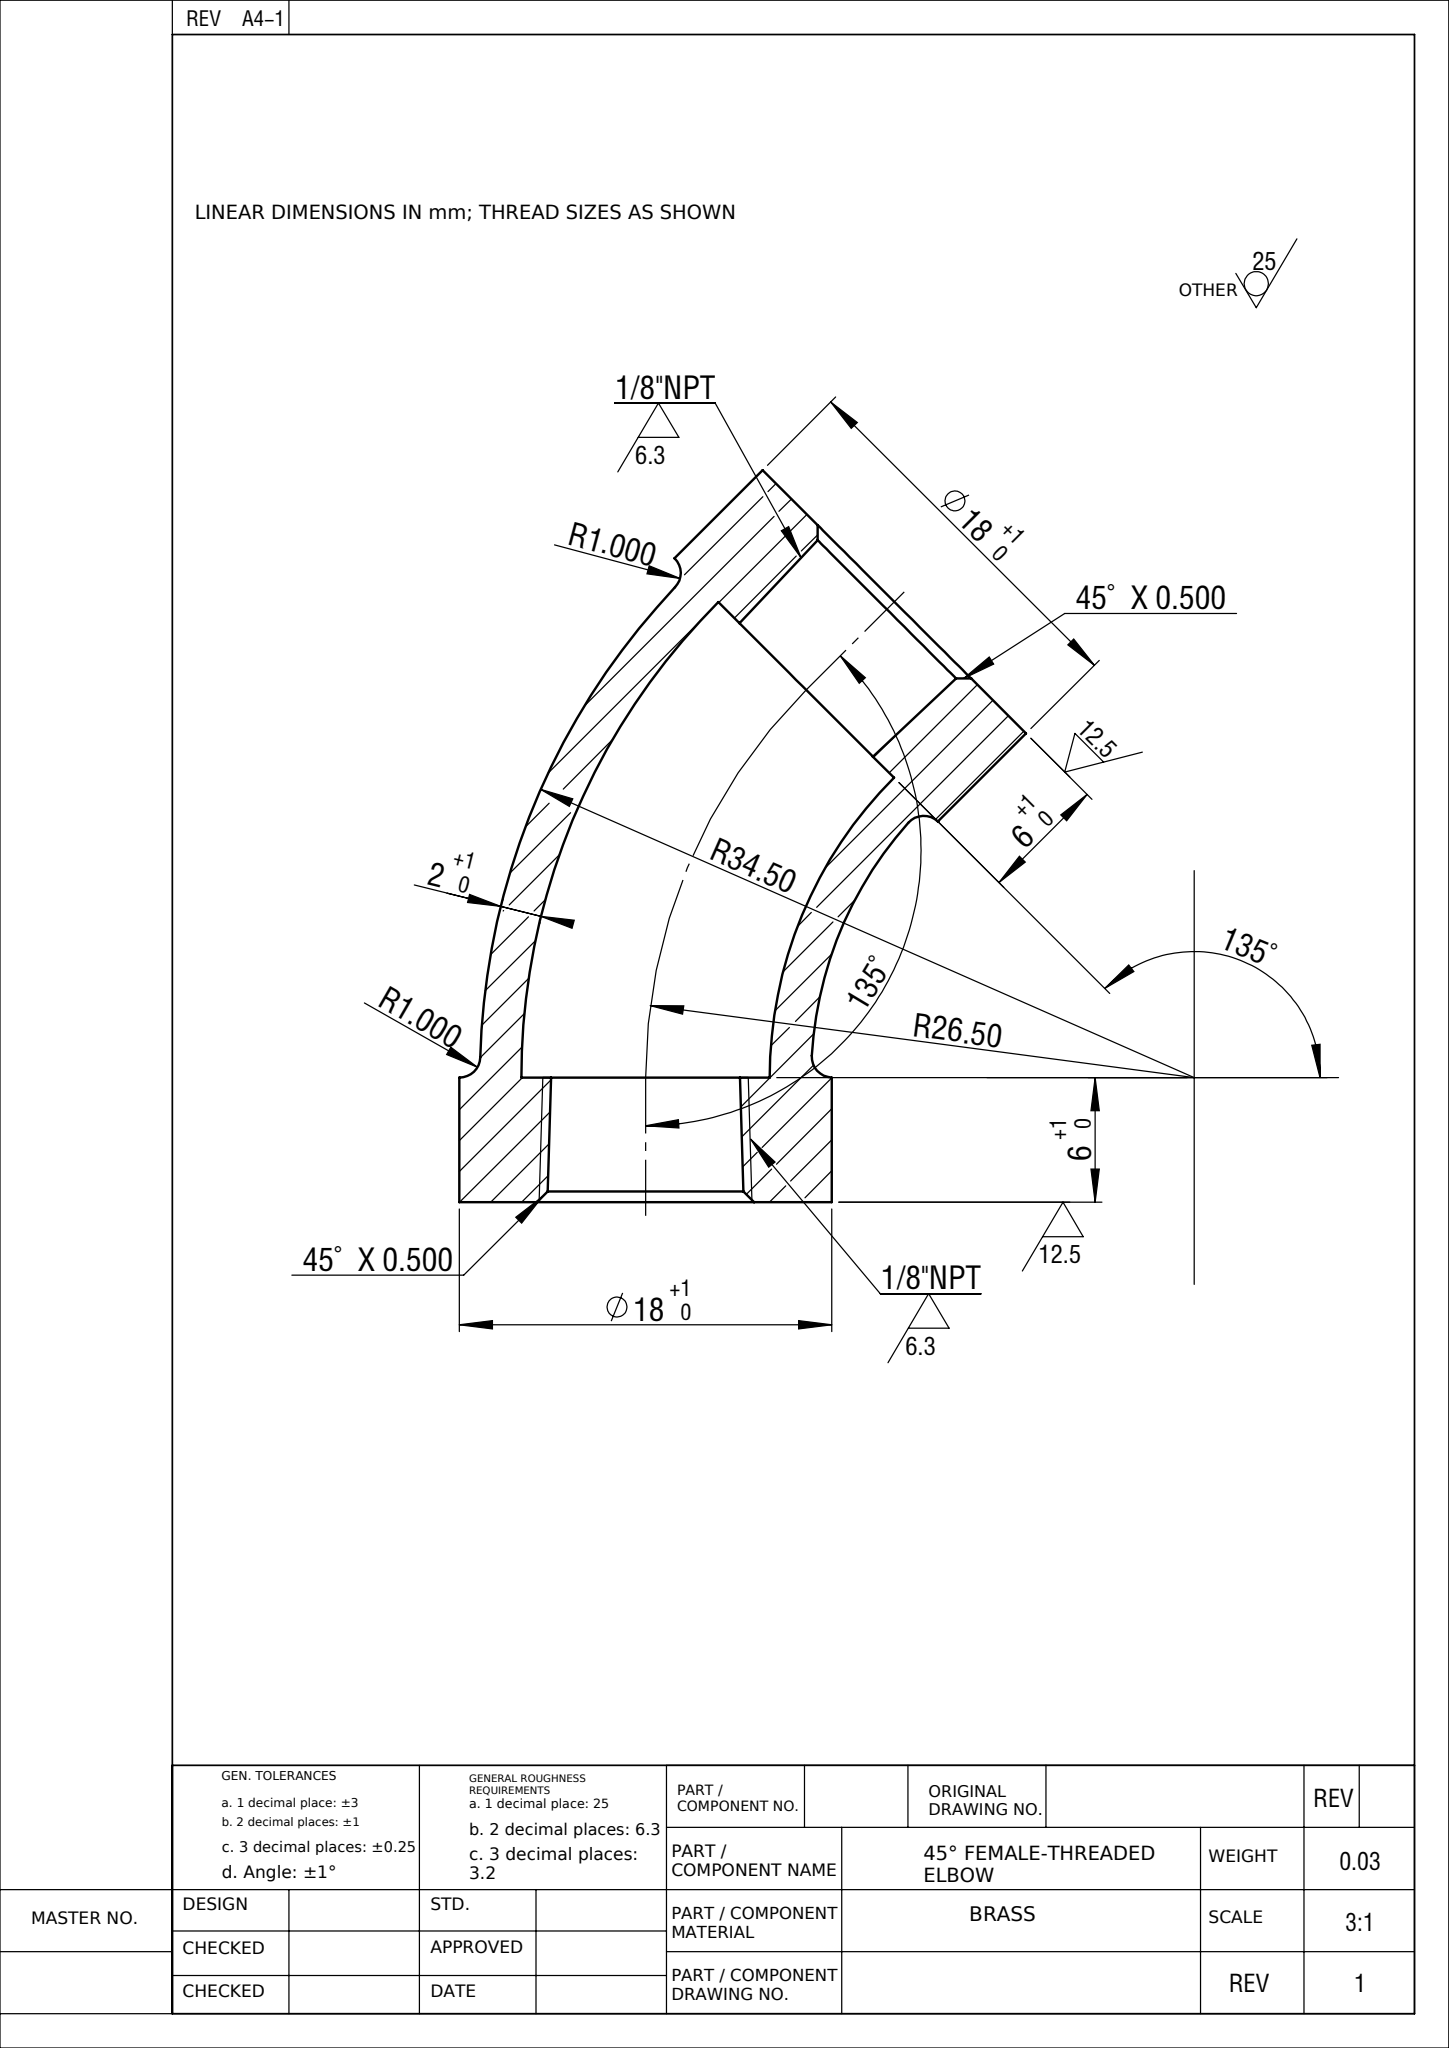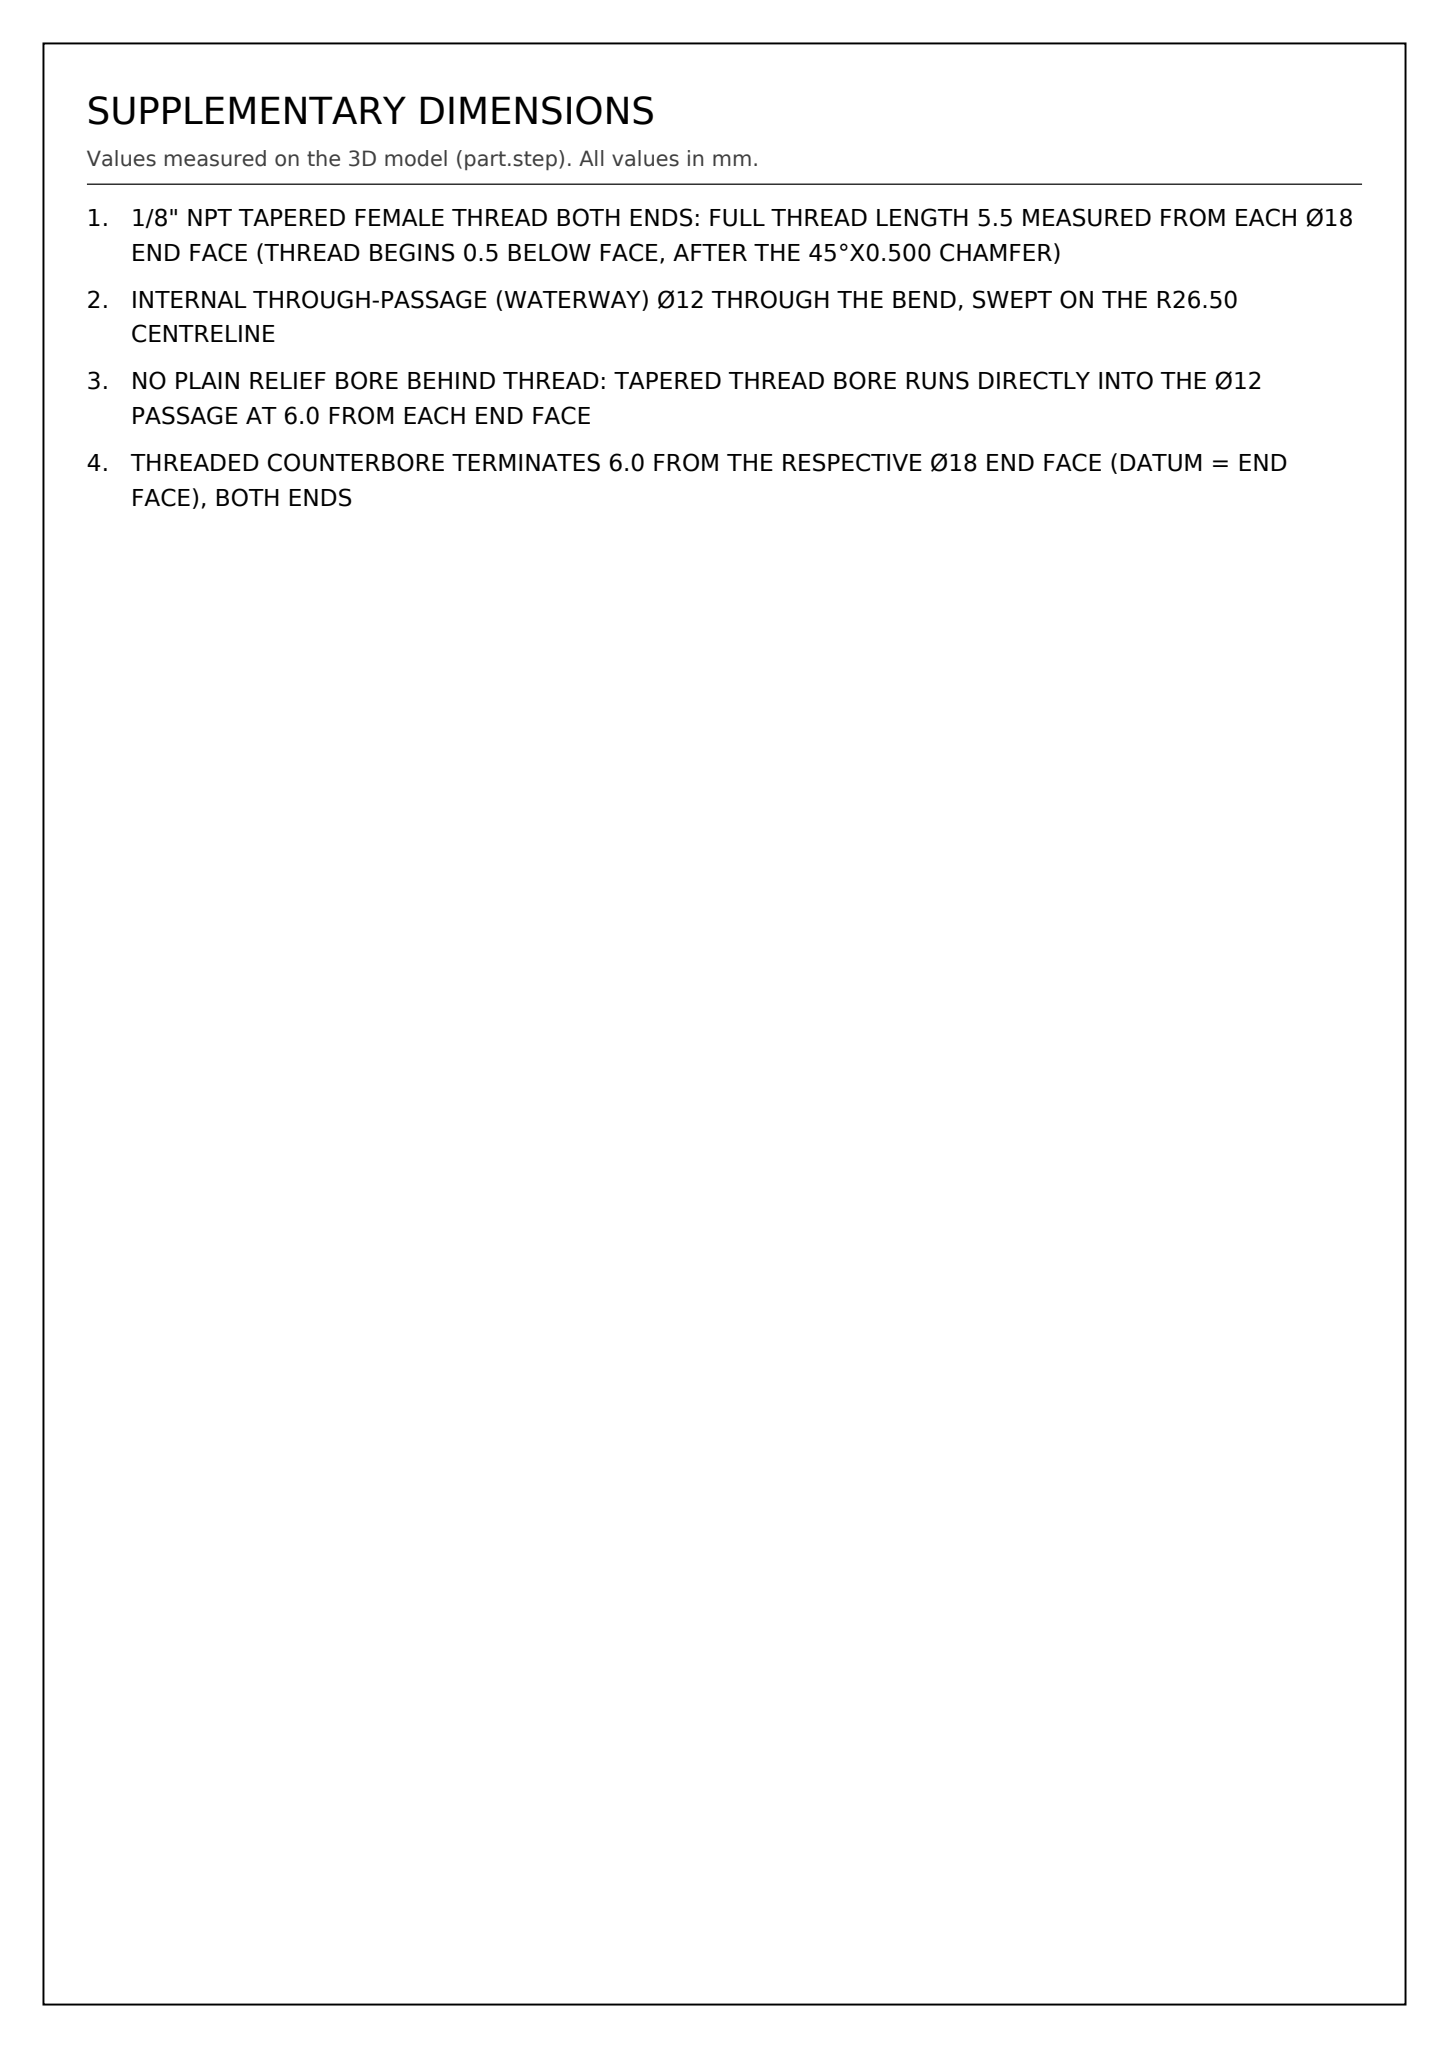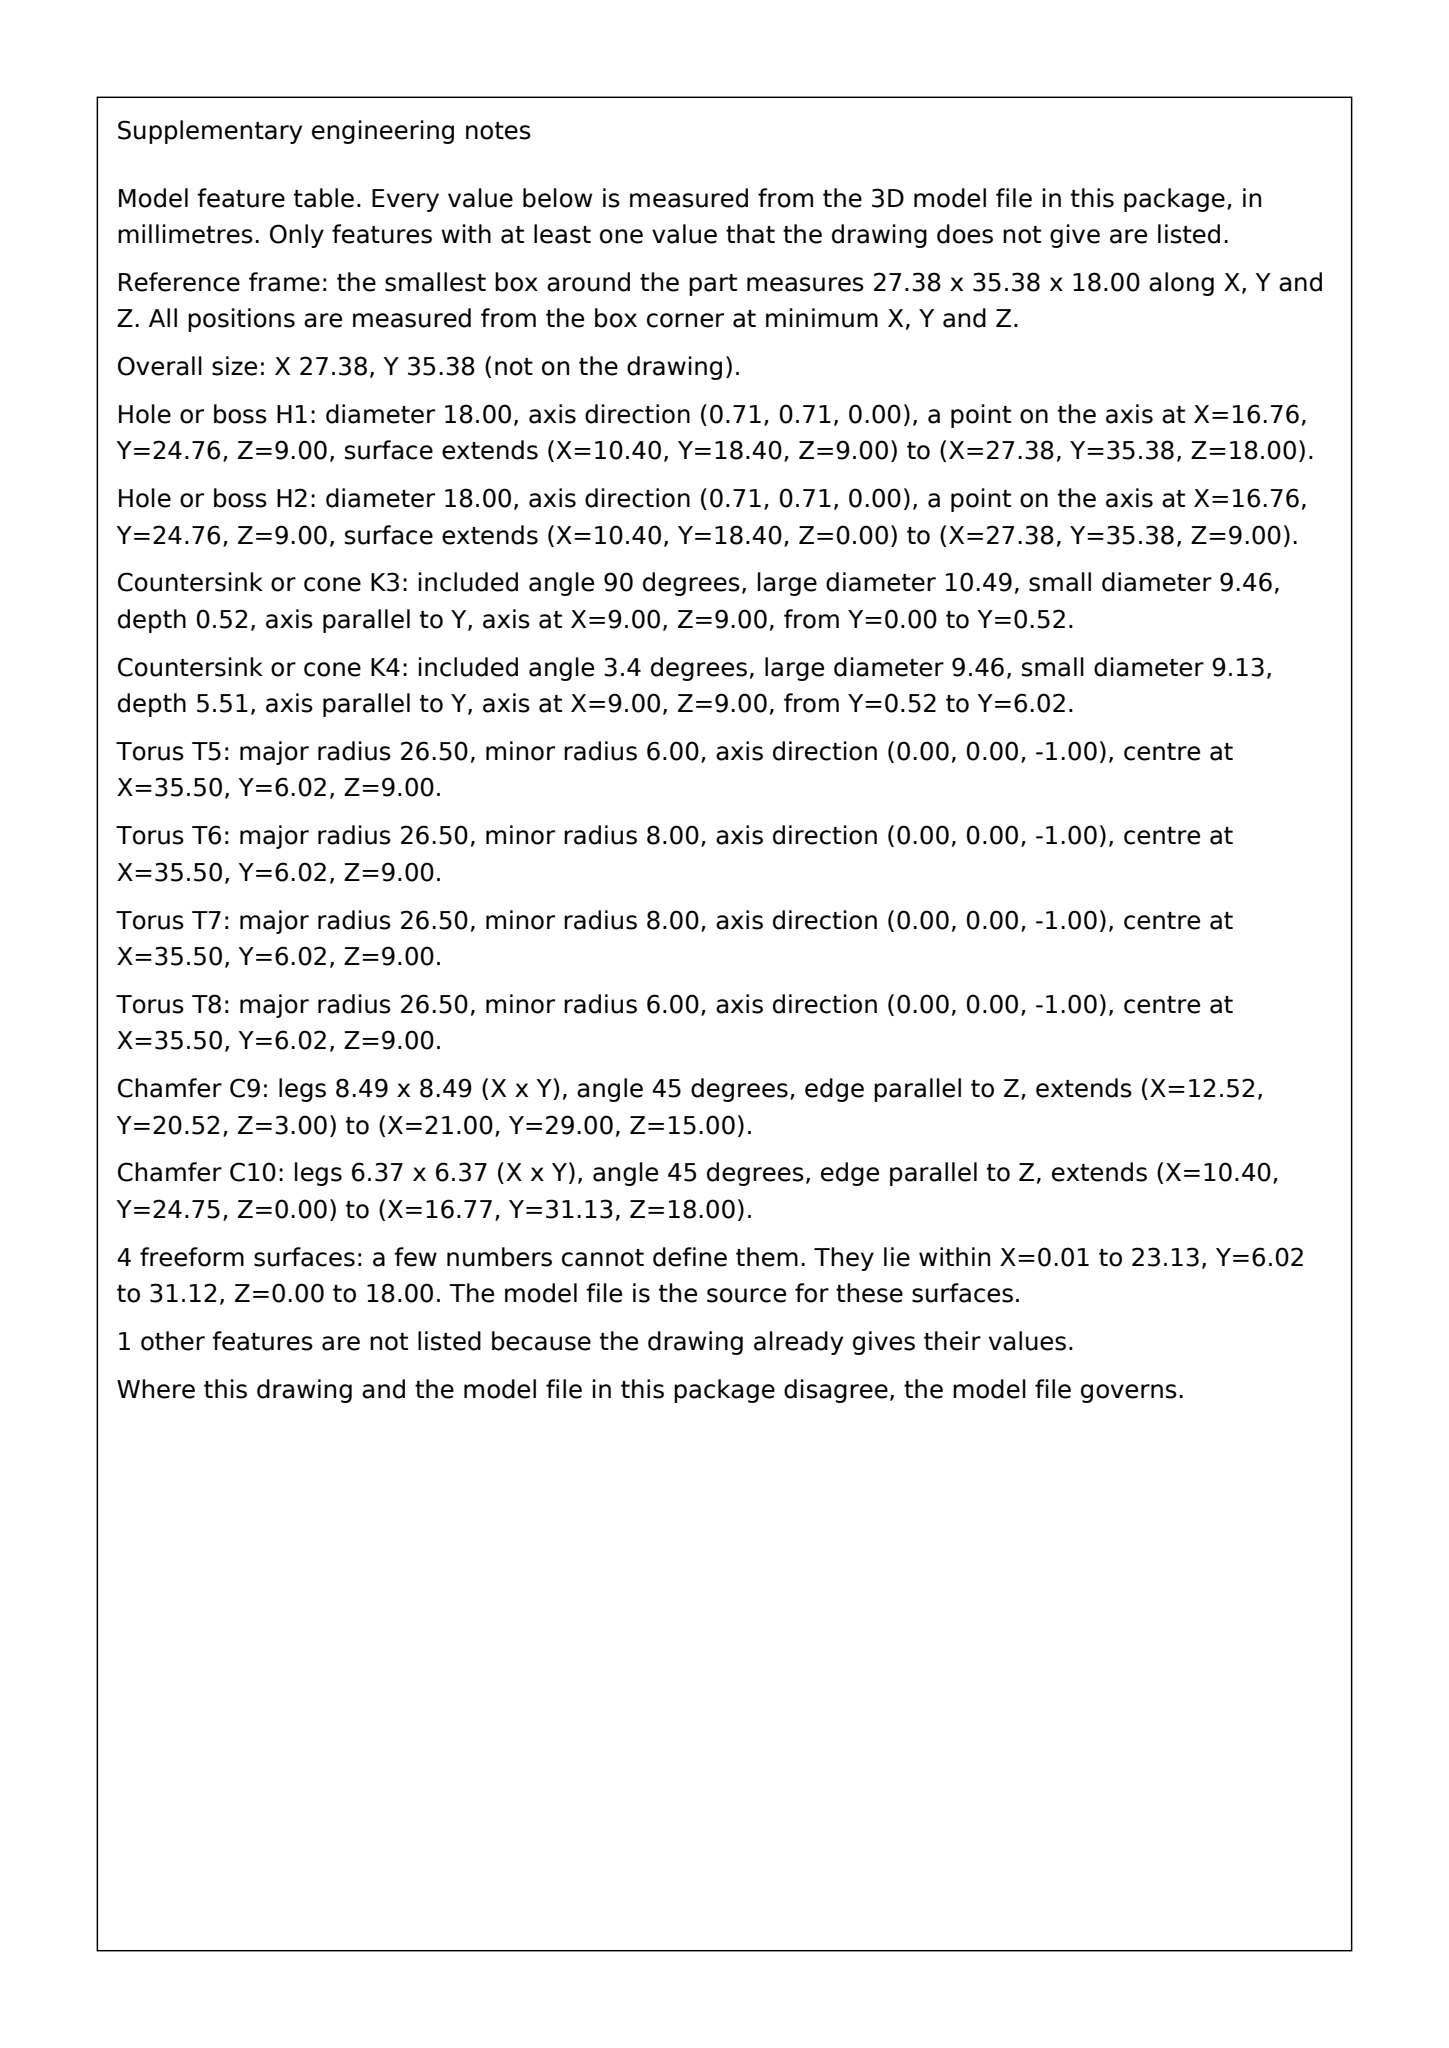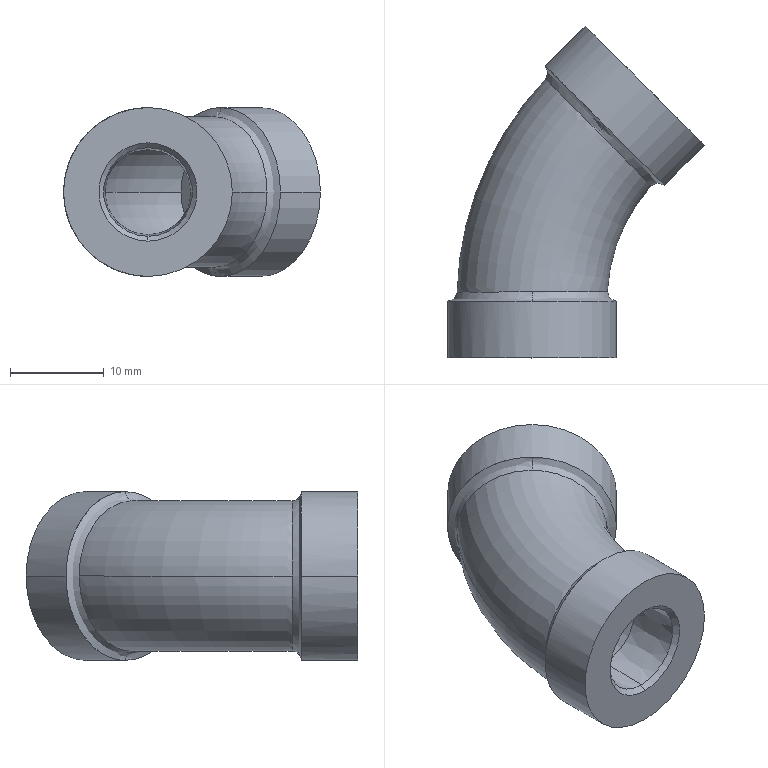Part | SolidWorks | mm | 1 solid | 26 faces | box 27.38 x 35.38 x 18 mm | volume 4091 mm3 | cone 8 | plane 6 | torus 4 | cylinder 4 | spline 4 | commonest cylinder face diameters 18 x4
Drawing notes:
1/8" NPT TAPERED FEMALE THREAD BOTH ENDS: FULL THREAD LENGTH 5.5 MEASURED FROM EACH Ø18 END FACE (THREAD BEGINS 0.5 BELOW FACE, AFTER THE 45°X0.500 CHAMFER) | from the solid: cones included_angle 3.4° ref_dia 9.49: pair at bbox_from [10.8,0.5,4.3] and [6.1,0.5,4.3], size [4.7,5.5,9.5] (y 0.5 to 6.0); matching inclined-end pair at [15.4,21.5,4.3] / [15.4,21.5,9.0]
INTERNAL THROUGH-PASSAGE (WATERWAY) Ø12 THROUGH THE BEND, SWEPT ON THE R26.50 CENTRELINE | from the solid: tori minor_r 6.0, major_r 26.5 (qty 2) = inner passage; outer tori minor_r 8.0, major_r 26.5 give the 2 wall thickness
NO PLAIN RELIEF BORE BEHIND THREAD: TAPERED THREAD BORE RUNS DIRECTLY INTO THE Ø12 PASSAGE AT 6.0 FROM EACH END FACE | from the solid: thread cones (3.4°) terminate at y=6.0; axis_plane normal y, offset 6.0, extent x [4.8,16.8] z [3.0,15.0], area 48
THREADED COUNTERBORE TERMINATES 6.0 FROM THE RESPECTIVE Ø18 END FACE (DATUM = END FACE), BOTH ENDS | from the solid: cylinder boss/shaft Ø18 y-axis from 0.0 to 6.0; inclined Ø18 boss from 12.2 to 29.2; axis_plane y offset 0.0 (end face) and y offset 6.0